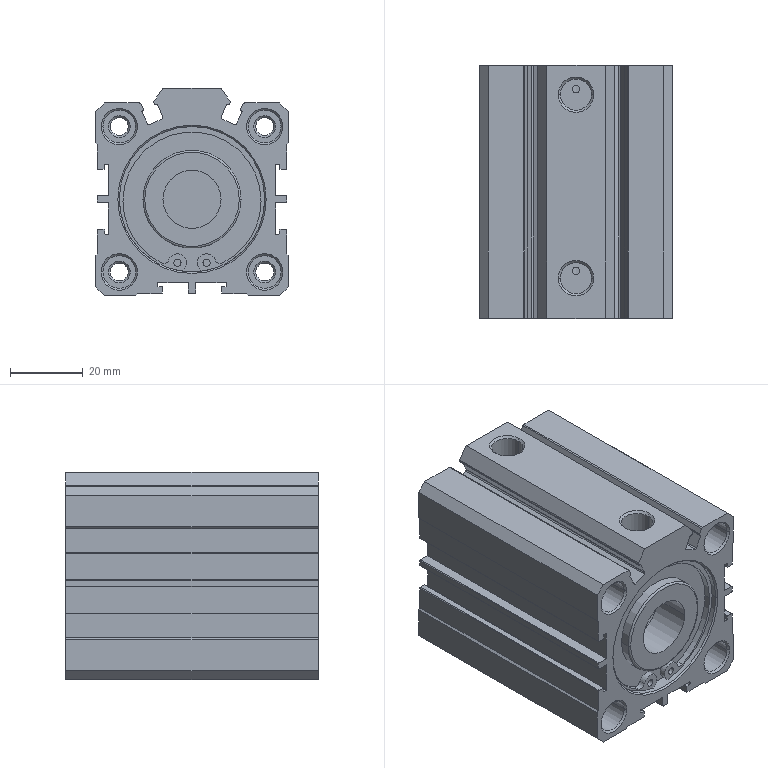Component | SolidWorks | ACQ40x30SB(0)+()-1_ACQS-40x3030_b-1 | 1 solid | 246 faces | volume 100833 mm3 | cylinder 108 | plane 92 | cone 44 | torus 2 | commonest cylinder face diameters 0.4 x35 9 x16 0.8 x15 2 x8 4.917 x8 40 x6 8.566 x4 38 x3